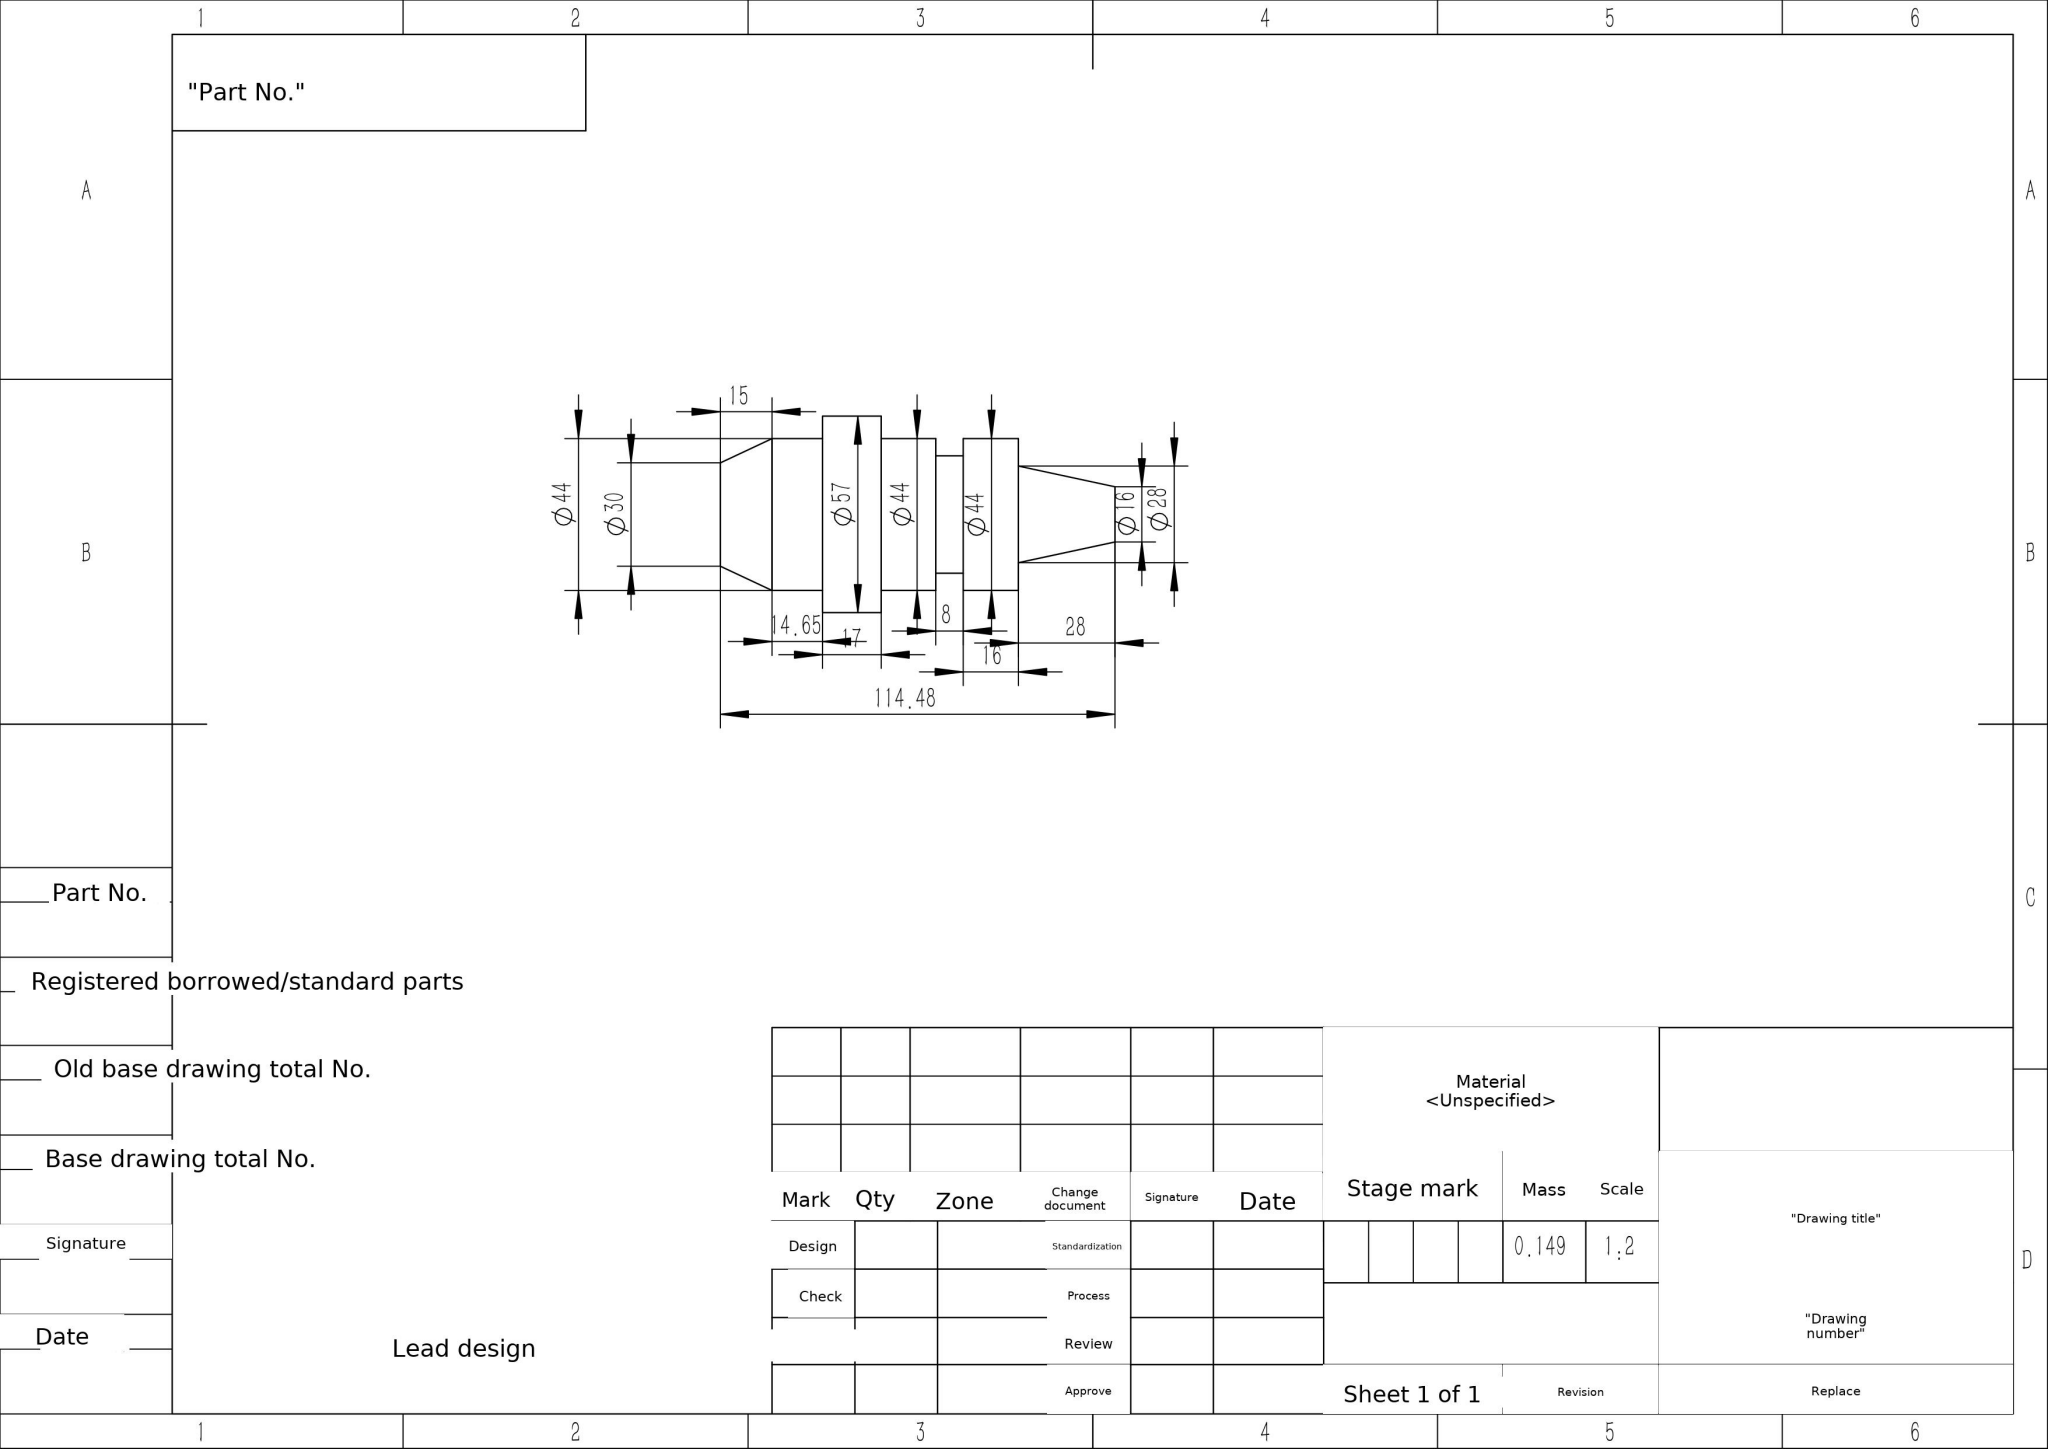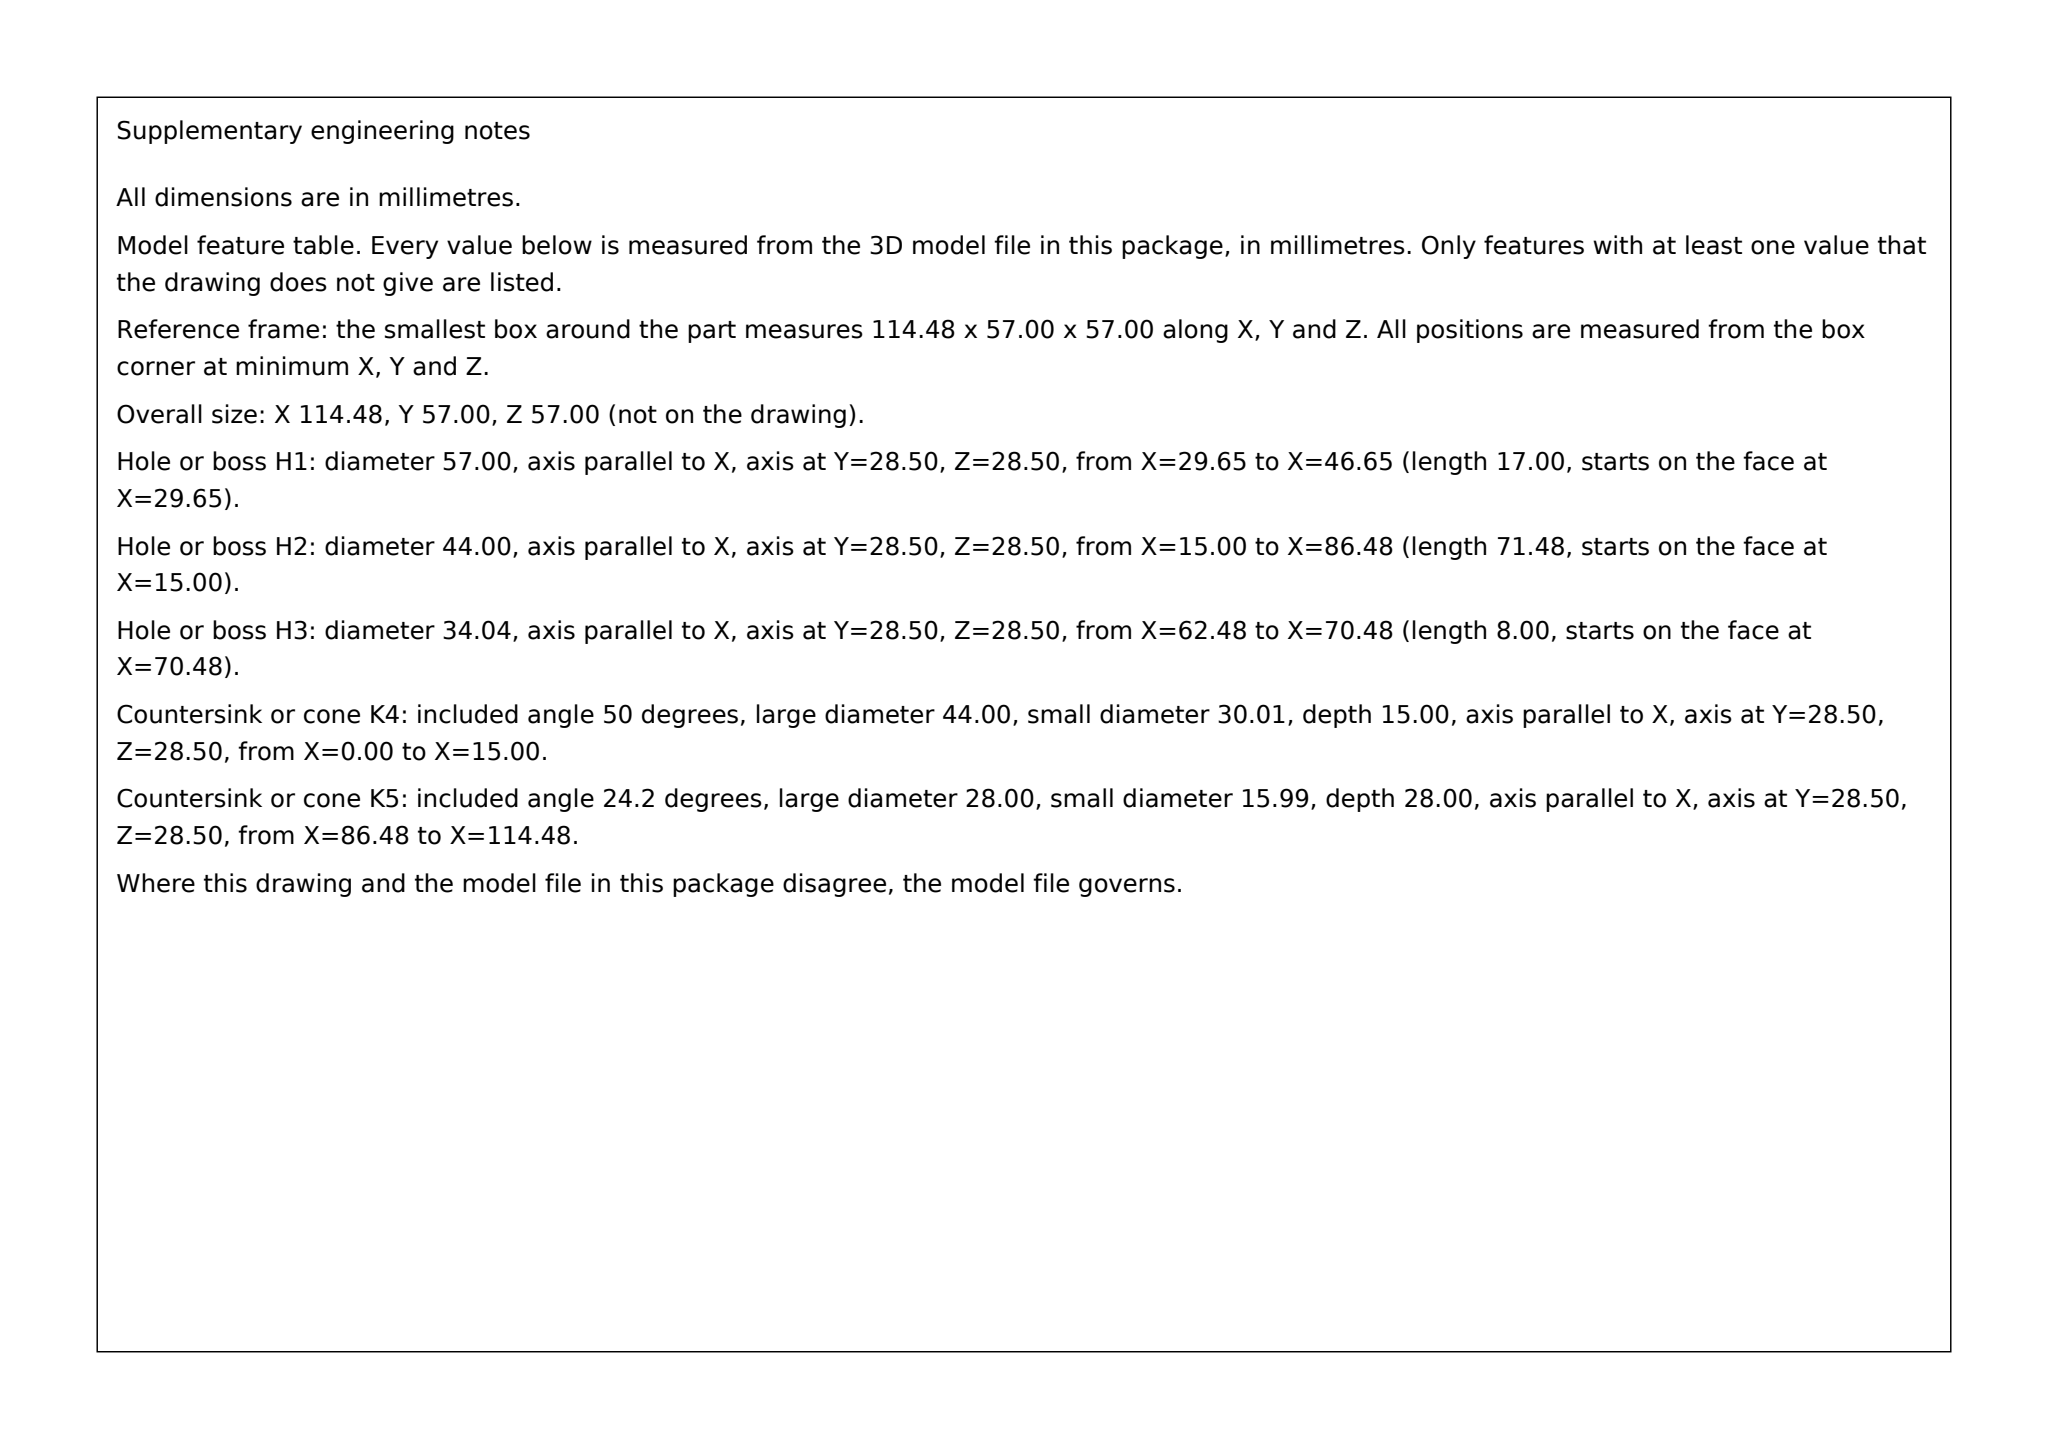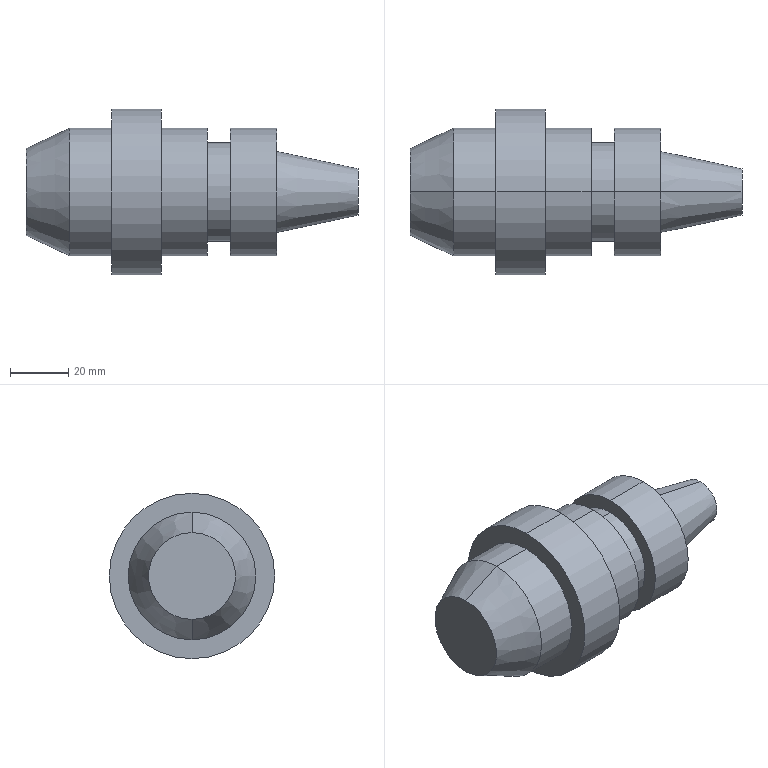Part | SolidWorks | mm | material <Unspecified> | 1 solid | 21 faces | box 114.48 x 57 x 57 mm | volume 148560 mm3 | cylinder 10 | plane 7 | cone 4 | commonest cylinder face diameters 44 x6 34.036 x2 57 x2
build123d program:
from build123d import *


with BuildPart() as part:
    # Sketch1 → Revolve1 (revolve)
    with BuildSketch(Plane.XY, mode=Mode.PRIVATE) as revolve1_sk:
        Polygon((0, 0), (0, 15), (15, 22), (29.653, 22), (29.653, 28.5), (46.653, 28.5), (46.653, 22), (62.479, 22), (62.479, 17.018), (70.479, 17.018), (70.479, 22), (86.479, 22), (86.479, 14), (114.479, 8), (114.479, 0), align=None)
    revolve(revolve1_sk.sketch.rotate(Axis((114.479, 0, 0), (-1, 0, 0)), 90), axis=Axis((114.479, 0, 0), (-1, 0, 0)))


solid = part.part
STEP:
#1=CARTESIAN_POINT('',(114.479,0.,-8.));
#2=VERTEX_POINT('',#1);
#3=CARTESIAN_POINT('',(114.479,0.,8.));
#4=VERTEX_POINT('',#3);
#5=CARTESIAN_POINT('',(114.479,0.,0.));
#6=DIRECTION('',(1.,0.,0.));
#7=DIRECTION('',(0.,0.,-1.));
#8=AXIS2_PLACEMENT_3D('',#5,#6,#7);
#9=CIRCLE('',#8,8.);
#10=EDGE_CURVE('',#2,#4,#9,.T.);
#11=ORIENTED_EDGE('',*,*,#10,.F.);
#12=CARTESIAN_POINT('',(86.479,0.,-14.));
#13=VERTEX_POINT('',#12);
#14=CARTESIAN_POINT('',(114.479,0.,-8.));
#15=DIRECTION('',(-0.9778,0.,-0.2095));
#16=VECTOR('',#15,1000.);
#17=LINE('',#14,#16);
#18=EDGE_CURVE('',#2,#13,#17,.T.);
#19=ORIENTED_EDGE('',*,*,#18,.T.);
#20=CARTESIAN_POINT('',(86.479,0.,14.));
#21=VERTEX_POINT('',#20);
#22=CARTESIAN_POINT('',(86.479,0.,0.));
#23=DIRECTION('',(1.,0.,0.));
#24=DIRECTION('',(0.,0.,-1.));
#25=AXIS2_PLACEMENT_3D('',#22,#23,#24);
#26=CIRCLE('',#25,14.);
#27=EDGE_CURVE('',#13,#21,#26,.T.);
#28=ORIENTED_EDGE('',*,*,#27,.T.);
#29=CARTESIAN_POINT('',(114.479,0.,8.));
#30=DIRECTION('',(-0.9778,0.,0.2095));
#31=VECTOR('',#30,1000.);
#32=LINE('',#29,#31);
#33=EDGE_CURVE('',#4,#21,#32,.T.);
#34=ORIENTED_EDGE('',*,*,#33,.F.);
#35=EDGE_LOOP('',(#11,#19,#28,#34));
#36=FACE_OUTER_BOUND('',#35,.T.);
#37=CARTESIAN_POINT('',(114.479,0.,0.));
#38=DIRECTION('',(-1.,0.,0.));
#39=DIRECTION('',(0.,0.,1.));
#40=AXIS2_PLACEMENT_3D('',#37,#38,#39);
#41=CONICAL_SURFACE('',#40,8.,0.2111);
#42=ADVANCED_FACE('',(#36),#41,.T.);
#43=CARTESIAN_POINT('',(70.479,0.,-22.));
#44=VERTEX_POINT('',#43);
#45=CARTESIAN_POINT('',(70.479,0.,22.));
#46=VERTEX_POINT('',#45);
#47=CARTESIAN_POINT('',(70.479,0.,0.));
#48=DIRECTION('',(1.,0.,0.));
#49=DIRECTION('',(0.,0.,-1.));
#50=AXIS2_PLACEMENT_3D('',#47,#48,#49);
#51=CIRCLE('',#50,22.);
#52=EDGE_CURVE('',#44,#46,#51,.T.);
#53=ORIENTED_EDGE('',*,*,#52,.T.);
#54=CARTESIAN_POINT('',(86.479,0.,22.));
#55=VERTEX_POINT('',#54);
#56=CARTESIAN_POINT('',(114.479,0.,22.));
#57=DIRECTION('',(1.,0.,0.));
#58=VECTOR('',#57,1000.);
#59=LINE('',#56,#58);
#60=EDGE_CURVE('',#46,#55,#59,.T.);
#61=ORIENTED_EDGE('',*,*,#60,.T.);
#62=CARTESIAN_POINT('',(86.479,0.,-22.));
#63=VERTEX_POINT('',#62);
#64=CARTESIAN_POINT('',(86.479,0.,0.));
#65=DIRECTION('',(1.,0.,0.));
#66=DIRECTION('',(0.,0.,-1.));
#67=AXIS2_PLACEMENT_3D('',#64,#65,#66);
#68=CIRCLE('',#67,22.);
#69=EDGE_CURVE('',#63,#55,#68,.T.);
#70=ORIENTED_EDGE('',*,*,#69,.F.);
#71=CARTESIAN_POINT('',(114.479,0.,-22.));
#72=DIRECTION('',(1.,0.,0.));
#73=VECTOR('',#72,1000.);
#74=LINE('',#71,#73);
#75=EDGE_CURVE('',#44,#63,#74,.T.);
#76=ORIENTED_EDGE('',*,*,#75,.F.);
#77=EDGE_LOOP('',(#53,#61,#70,#76));
#78=FACE_OUTER_BOUND('',#77,.T.);
#79=CARTESIAN_POINT('',(114.479,0.,0.));
#80=DIRECTION('',(1.,0.,0.));
#81=DIRECTION('',(0.,0.,-1.));
#82=AXIS2_PLACEMENT_3D('',#79,#80,#81);
#83=CYLINDRICAL_SURFACE('',#82,22.);
#84=ADVANCED_FACE('',(#78),#83,.T.);
#85=CARTESIAN_POINT('',(62.479,0.,-17.018));
#86=VERTEX_POINT('',#85);
#87=CARTESIAN_POINT('',(62.479,0.,17.018));
#88=VERTEX_POINT('',#87);
#89=CARTESIAN_POINT('',(62.479,0.,0.));
#90=DIRECTION('',(1.,0.,0.));
#91=DIRECTION('',(0.,0.,-1.));
#92=AXIS2_PLACEMENT_3D('',#89,#90,#91);
#93=CIRCLE('',#92,17.018);
#94=EDGE_CURVE('',#86,#88,#93,.T.);
#95=ORIENTED_EDGE('',*,*,#94,.T.);
#96=CARTESIAN_POINT('',(70.479,0.,17.018));
#97=VERTEX_POINT('',#96);
#98=CARTESIAN_POINT('',(114.479,0.,17.018));
#99=DIRECTION('',(1.,0.,0.));
#100=VECTOR('',#99,1000.);
#101=LINE('',#98,#100);
#102=EDGE_CURVE('',#88,#97,#101,.T.);
#103=ORIENTED_EDGE('',*,*,#102,.T.);
#104=CARTESIAN_POINT('',(70.479,0.,-17.018));
#105=VERTEX_POINT('',#104);
#106=CARTESIAN_POINT('',(70.479,0.,0.));
#107=DIRECTION('',(1.,0.,0.));
#108=DIRECTION('',(0.,0.,-1.));
#109=AXIS2_PLACEMENT_3D('',#106,#107,#108);
#110=CIRCLE('',#109,17.018);
#111=EDGE_CURVE('',#105,#97,#110,.T.);
#112=ORIENTED_EDGE('',*,*,#111,.F.);
#113=CARTESIAN_POINT('',(114.479,0.,-17.018));
#114=DIRECTION('',(1.,0.,0.));
#115=VECTOR('',#114,1000.);
#116=LINE('',#113,#115);
#117=EDGE_CURVE('',#86,#105,#116,.T.);
#118=ORIENTED_EDGE('',*,*,#117,.F.);
#119=EDGE_LOOP('',(#95,#103,#112,#118));
#120=FACE_OUTER_BOUND('',#119,.T.);
#121=CARTESIAN_POINT('',(114.479,0.,0.));
#122=DIRECTION('',(1.,0.,0.));
#123=DIRECTION('',(0.,0.,-1.));
#124=AXIS2_PLACEMENT_3D('',#121,#122,#123);
#125=CYLINDRICAL_SURFACE('',#124,17.018);
#126=ADVANCED_FACE('',(#120),#125,.T.);
#127=CARTESIAN_POINT('',(46.653,0.,-22.));
#128=VERTEX_POINT('',#127);
#129=CARTESIAN_POINT('',(46.653,0.,22.));
#130=VERTEX_POINT('',#129);
#131=CARTESIAN_POINT('',(46.653,0.,0.));
#132=DIRECTION('',(1.,0.,0.));
#133=DIRECTION('',(0.,0.,-1.));
#134=AXIS2_PLACEMENT_3D('',#131,#132,#133);
#135=CIRCLE('',#134,22.);
#136=EDGE_CURVE('',#128,#130,#135,.T.);
#137=ORIENTED_EDGE('',*,*,#136,.T.);
#138=CARTESIAN_POINT('',(62.479,0.,22.));
#139=VERTEX_POINT('',#138);
#140=CARTESIAN_POINT('',(114.479,0.,22.));
#141=DIRECTION('',(1.,0.,0.));
#142=VECTOR('',#141,1000.);
#143=LINE('',#140,#142);
#144=EDGE_CURVE('',#130,#139,#143,.T.);
#145=ORIENTED_EDGE('',*,*,#144,.T.);
#146=CARTESIAN_POINT('',(62.479,0.,-22.));
#147=VERTEX_POINT('',#146);
#148=CARTESIAN_POINT('',(62.479,0.,0.));
#149=DIRECTION('',(1.,0.,0.));
#150=DIRECTION('',(0.,0.,-1.));
#151=AXIS2_PLACEMENT_3D('',#148,#149,#150);
#152=CIRCLE('',#151,22.);
#153=EDGE_CURVE('',#147,#139,#152,.T.);
#154=ORIENTED_EDGE('',*,*,#153,.F.);
#155=CARTESIAN_POINT('',(114.479,0.,-22.));
#156=DIRECTION('',(1.,0.,0.));
#157=VECTOR('',#156,1000.);
#158=LINE('',#155,#157);
#159=EDGE_CURVE('',#128,#147,#158,.T.);
#160=ORIENTED_EDGE('',*,*,#159,.F.);
#161=EDGE_LOOP('',(#137,#145,#154,#160));
#162=FACE_OUTER_BOUND('',#161,.T.);
#163=CARTESIAN_POINT('',(114.479,0.,0.));
#164=DIRECTION('',(1.,0.,0.));
#165=DIRECTION('',(0.,0.,-1.));
#166=AXIS2_PLACEMENT_3D('',#163,#164,#165);
#167=CYLINDRICAL_SURFACE('',#166,22.);
#168=ADVANCED_FACE('',(#162),#167,.T.);
#169=CARTESIAN_POINT('',(29.653,0.,-28.5));
#170=VERTEX_POINT('',#169);
#171=CARTESIAN_POINT('',(29.653,0.,28.5));
#172=VERTEX_POINT('',#171);
#173=CARTESIAN_POINT('',(29.653,0.,0.));
#174=DIRECTION('',(1.,0.,0.));
#175=DIRECTION('',(0.,0.,-1.));
#176=AXIS2_PLACEMENT_3D('',#173,#174,#175);
#177=CIRCLE('',#176,28.5);
#178=EDGE_CURVE('',#170,#172,#177,.T.);
#179=ORIENTED_EDGE('',*,*,#178,.T.);
#180=CARTESIAN_POINT('',(46.653,0.,28.5));
#181=VERTEX_POINT('',#180);
#182=CARTESIAN_POINT('',(114.479,0.,28.5));
#183=DIRECTION('',(1.,0.,0.));
#184=VECTOR('',#183,1000.);
#185=LINE('',#182,#184);
#186=EDGE_CURVE('',#172,#181,#185,.T.);
#187=ORIENTED_EDGE('',*,*,#186,.T.);
#188=CARTESIAN_POINT('',(46.653,0.,-28.5));
#189=VERTEX_POINT('',#188);
#190=CARTESIAN_POINT('',(46.653,0.,0.));
#191=DIRECTION('',(1.,0.,0.));
#192=DIRECTION('',(0.,0.,-1.));
#193=AXIS2_PLACEMENT_3D('',#190,#191,#192);
#194=CIRCLE('',#193,28.5);
#195=EDGE_CURVE('',#189,#181,#194,.T.);
#196=ORIENTED_EDGE('',*,*,#195,.F.);
#197=CARTESIAN_POINT('',(114.479,0.,-28.5));
#198=DIRECTION('',(1.,0.,0.));
#199=VECTOR('',#198,1000.);
#200=LINE('',#197,#199);
#201=EDGE_CURVE('',#170,#189,#200,.T.);
#202=ORIENTED_EDGE('',*,*,#201,.F.);
#203=EDGE_LOOP('',(#179,#187,#196,#202));
#204=FACE_OUTER_BOUND('',#203,.T.);
#205=CARTESIAN_POINT('',(114.479,0.,0.));
#206=DIRECTION('',(1.,0.,0.));
#207=DIRECTION('',(0.,0.,-1.));
#208=AXIS2_PLACEMENT_3D('',#205,#206,#207);
#209=CYLINDRICAL_SURFACE('',#208,28.5);
#210=ADVANCED_FACE('',(#204),#209,.T.);
#211=CARTESIAN_POINT('',(15.,0.,-22.));
#212=VERTEX_POINT('',#211);
#213=CARTESIAN_POINT('',(15.,0.,22.));
#214=VERTEX_POINT('',#213);
#215=CARTESIAN_POINT('',(15.,0.,0.));
#216=DIRECTION('',(1.,0.,0.));
#217=DIRECTION('',(0.,0.,-1.));
#218=AXIS2_PLACEMENT_3D('',#215,#216,#217);
#219=CIRCLE('',#218,22.);
#220=EDGE_CURVE('',#212,#214,#219,.T.);
#221=ORIENTED_EDGE('',*,*,#220,.T.);
#222=CARTESIAN_POINT('',(29.653,0.,22.));
#223=VERTEX_POINT('',#222);
#224=CARTESIAN_POINT('',(114.479,0.,22.));
#225=DIRECTION('',(1.,0.,0.));
#226=VECTOR('',#225,1000.);
#227=LINE('',#224,#226);
#228=EDGE_CURVE('',#214,#223,#227,.T.);
#229=ORIENTED_EDGE('',*,*,#228,.T.);
#230=CARTESIAN_POINT('',(29.653,0.,-22.));
#231=VERTEX_POINT('',#230);
#232=CARTESIAN_POINT('',(29.653,0.,0.));
#233=DIRECTION('',(1.,0.,0.));
#234=DIRECTION('',(0.,0.,-1.));
#235=AXIS2_PLACEMENT_3D('',#232,#233,#234);
#236=CIRCLE('',#235,22.);
#237=EDGE_CURVE('',#231,#223,#236,.T.);
#238=ORIENTED_EDGE('',*,*,#237,.F.);
#239=CARTESIAN_POINT('',(114.479,0.,-22.));
#240=DIRECTION('',(1.,0.,0.));
#241=VECTOR('',#240,1000.);
#242=LINE('',#239,#241);
#243=EDGE_CURVE('',#212,#231,#242,.T.);
#244=ORIENTED_EDGE('',*,*,#243,.F.);
#245=EDGE_LOOP('',(#221,#229,#238,#244));
#246=FACE_OUTER_BOUND('',#245,.T.);
#247=CARTESIAN_POINT('',(114.479,0.,0.));
#248=DIRECTION('',(1.,0.,0.));
#249=DIRECTION('',(0.,0.,-1.));
#250=AXIS2_PLACEMENT_3D('',#247,#248,#249);
#251=CYLINDRICAL_SURFACE('',#250,22.);
#252=ADVANCED_FACE('',(#246),#251,.T.);
#253=CARTESIAN_POINT('',(0.,0.,-15.));
#254=VERTEX_POINT('',#253);
#255=CARTESIAN_POINT('',(0.,0.,15.));
#256=VERTEX_POINT('',#255);
#257=CARTESIAN_POINT('',(0.,0.,0.));
#258=DIRECTION('',(1.,0.,0.));
#259=DIRECTION('',(0.,0.,-1.));
#260=AXIS2_PLACEMENT_3D('',#257,#258,#259);
#261=CIRCLE('',#260,15.);
#262=EDGE_CURVE('',#254,#256,#261,.T.);
#263=ORIENTED_EDGE('',*,*,#262,.T.);
#264=CARTESIAN_POINT('',(15.,0.,22.));
#265=DIRECTION('',(0.9062,0.,0.4229));
#266=VECTOR('',#265,1000.);
#267=LINE('',#264,#266);
#268=EDGE_CURVE('',#256,#214,#267,.T.);
#269=ORIENTED_EDGE('',*,*,#268,.T.);
#270=ORIENTED_EDGE('',*,*,#220,.F.);
#271=CARTESIAN_POINT('',(15.,0.,-22.));
#272=DIRECTION('',(0.9062,0.,-0.4229));
#273=VECTOR('',#272,1000.);
#274=LINE('',#271,#273);
#275=EDGE_CURVE('',#254,#212,#274,.T.);
#276=ORIENTED_EDGE('',*,*,#275,.F.);
#277=EDGE_LOOP('',(#263,#269,#270,#276));
#278=FACE_OUTER_BOUND('',#277,.T.);
#279=CARTESIAN_POINT('',(15.,0.,0.));
#280=DIRECTION('',(1.,0.,0.));
#281=DIRECTION('',(0.,0.,-1.));
#282=AXIS2_PLACEMENT_3D('',#279,#280,#281);
#283=CONICAL_SURFACE('',#282,22.,0.4366);
#284=ADVANCED_FACE('',(#278),#283,.T.);
#285=ORIENTED_EDGE('',*,*,#262,.F.);
#286=CARTESIAN_POINT('',(0.,0.,0.));
#287=DIRECTION('',(1.,0.,0.));
#288=DIRECTION('',(0.,0.,-1.));
#289=AXIS2_PLACEMENT_3D('',#286,#287,#288);
#290=CIRCLE('',#289,15.);
#291=EDGE_CURVE('',#256,#254,#290,.T.);
#292=ORIENTED_EDGE('',*,*,#291,.F.);
#293=EDGE_LOOP('',(#285,#292));
#294=FACE_OUTER_BOUND('',#293,.T.);
#295=CARTESIAN_POINT('',(0.,0.,0.));
#296=DIRECTION('',(-1.,0.,0.));
#297=DIRECTION('',(0.,0.,1.));
#298=AXIS2_PLACEMENT_3D('',#295,#296,#297);
#299=PLANE('',#298);
#300=ADVANCED_FACE('',(#294),#299,.T.);
#301=ORIENTED_EDGE('',*,*,#268,.F.);
#302=ORIENTED_EDGE('',*,*,#291,.T.);
#303=ORIENTED_EDGE('',*,*,#275,.T.);
#304=CARTESIAN_POINT('',(15.,0.,0.));
#305=DIRECTION('',(1.,0.,0.));
#306=DIRECTION('',(0.,0.,-1.));
#307=AXIS2_PLACEMENT_3D('',#304,#305,#306);
#308=CIRCLE('',#307,22.);
#309=EDGE_CURVE('',#214,#212,#308,.T.);
#310=ORIENTED_EDGE('',*,*,#309,.F.);
#311=EDGE_LOOP('',(#301,#302,#303,#310));
#312=FACE_OUTER_BOUND('',#311,.T.);
#313=CARTESIAN_POINT('',(15.,0.,0.));
#314=DIRECTION('',(1.,0.,0.));
#315=DIRECTION('',(0.,0.,-1.));
#316=AXIS2_PLACEMENT_3D('',#313,#314,#315);
#317=CONICAL_SURFACE('',#316,22.,0.4366);
#318=ADVANCED_FACE('',(#312),#317,.T.);
#319=ORIENTED_EDGE('',*,*,#228,.F.);
#320=ORIENTED_EDGE('',*,*,#309,.T.);
#321=ORIENTED_EDGE('',*,*,#243,.T.);
#322=CARTESIAN_POINT('',(29.653,0.,0.));
#323=DIRECTION('',(1.,0.,0.));
#324=DIRECTION('',(0.,0.,-1.));
#325=AXIS2_PLACEMENT_3D('',#322,#323,#324);
#326=CIRCLE('',#325,22.);
#327=EDGE_CURVE('',#223,#231,#326,.T.);
#328=ORIENTED_EDGE('',*,*,#327,.F.);
#329=EDGE_LOOP('',(#319,#320,#321,#328));
#330=FACE_OUTER_BOUND('',#329,.T.);
#331=CARTESIAN_POINT('',(114.479,0.,0.));
#332=DIRECTION('',(1.,0.,0.));
#333=DIRECTION('',(0.,0.,-1.));
#334=AXIS2_PLACEMENT_3D('',#331,#332,#333);
#335=CYLINDRICAL_SURFACE('',#334,22.);
#336=ADVANCED_FACE('',(#330),#335,.T.);
#337=ORIENTED_EDGE('',*,*,#237,.T.);
#338=ORIENTED_EDGE('',*,*,#327,.T.);
#339=EDGE_LOOP('',(#337,#338));
#340=FACE_BOUND('',#339,.T.);
#341=ORIENTED_EDGE('',*,*,#178,.F.);
#342=CARTESIAN_POINT('',(29.653,0.,0.));
#343=DIRECTION('',(1.,0.,0.));
#344=DIRECTION('',(0.,0.,-1.));
#345=AXIS2_PLACEMENT_3D('',#342,#343,#344);
#346=CIRCLE('',#345,28.5);
#347=EDGE_CURVE('',#172,#170,#346,.T.);
#348=ORIENTED_EDGE('',*,*,#347,.F.);
#349=EDGE_LOOP('',(#341,#348));
#350=FACE_OUTER_BOUND('',#349,.T.);
#351=CARTESIAN_POINT('',(29.653,22.,0.));
#352=DIRECTION('',(-1.,0.,0.));
#353=DIRECTION('',(0.,0.,1.));
#354=AXIS2_PLACEMENT_3D('',#351,#352,#353);
#355=PLANE('',#354);
#356=ADVANCED_FACE('',(#340,#350),#355,.T.);
#357=ORIENTED_EDGE('',*,*,#186,.F.);
#358=ORIENTED_EDGE('',*,*,#347,.T.);
#359=ORIENTED_EDGE('',*,*,#201,.T.);
#360=CARTESIAN_POINT('',(46.653,0.,0.));
#361=DIRECTION('',(1.,0.,0.));
#362=DIRECTION('',(0.,0.,-1.));
#363=AXIS2_PLACEMENT_3D('',#360,#361,#362);
#364=CIRCLE('',#363,28.5);
#365=EDGE_CURVE('',#181,#189,#364,.T.);
#366=ORIENTED_EDGE('',*,*,#365,.F.);
#367=EDGE_LOOP('',(#357,#358,#359,#366));
#368=FACE_OUTER_BOUND('',#367,.T.);
#369=CARTESIAN_POINT('',(114.479,0.,0.));
#370=DIRECTION('',(1.,0.,0.));
#371=DIRECTION('',(0.,0.,-1.));
#372=AXIS2_PLACEMENT_3D('',#369,#370,#371);
#373=CYLINDRICAL_SURFACE('',#372,28.5);
#374=ADVANCED_FACE('',(#368),#373,.T.);
#375=ORIENTED_EDGE('',*,*,#195,.T.);
#376=ORIENTED_EDGE('',*,*,#365,.T.);
#377=EDGE_LOOP('',(#375,#376));
#378=FACE_OUTER_BOUND('',#377,.T.);
#379=ORIENTED_EDGE('',*,*,#136,.F.);
#380=CARTESIAN_POINT('',(46.653,0.,0.));
#381=DIRECTION('',(1.,0.,0.));
#382=DIRECTION('',(0.,0.,-1.));
#383=AXIS2_PLACEMENT_3D('',#380,#381,#382);
#384=CIRCLE('',#383,22.);
#385=EDGE_CURVE('',#130,#128,#384,.T.);
#386=ORIENTED_EDGE('',*,*,#385,.F.);
#387=EDGE_LOOP('',(#379,#386));
#388=FACE_BOUND('',#387,.T.);
#389=CARTESIAN_POINT('',(46.653,28.5,0.));
#390=DIRECTION('',(1.,0.,0.));
#391=DIRECTION('',(0.,0.,-1.));
#392=AXIS2_PLACEMENT_3D('',#389,#390,#391);
#393=PLANE('',#392);
#394=ADVANCED_FACE('',(#378,#388),#393,.T.);
#395=ORIENTED_EDGE('',*,*,#144,.F.);
#396=ORIENTED_EDGE('',*,*,#385,.T.);
#397=ORIENTED_EDGE('',*,*,#159,.T.);
#398=CARTESIAN_POINT('',(62.479,0.,0.));
#399=DIRECTION('',(1.,0.,0.));
#400=DIRECTION('',(0.,0.,-1.));
#401=AXIS2_PLACEMENT_3D('',#398,#399,#400);
#402=CIRCLE('',#401,22.);
#403=EDGE_CURVE('',#139,#147,#402,.T.);
#404=ORIENTED_EDGE('',*,*,#403,.F.);
#405=EDGE_LOOP('',(#395,#396,#397,#404));
#406=FACE_OUTER_BOUND('',#405,.T.);
#407=CARTESIAN_POINT('',(114.479,0.,0.));
#408=DIRECTION('',(1.,0.,0.));
#409=DIRECTION('',(0.,0.,-1.));
#410=AXIS2_PLACEMENT_3D('',#407,#408,#409);
#411=CYLINDRICAL_SURFACE('',#410,22.);
#412=ADVANCED_FACE('',(#406),#411,.T.);
#413=ORIENTED_EDGE('',*,*,#153,.T.);
#414=ORIENTED_EDGE('',*,*,#403,.T.);
#415=EDGE_LOOP('',(#413,#414));
#416=FACE_OUTER_BOUND('',#415,.T.);
#417=ORIENTED_EDGE('',*,*,#94,.F.);
#418=CARTESIAN_POINT('',(62.479,0.,0.));
#419=DIRECTION('',(1.,0.,0.));
#420=DIRECTION('',(0.,0.,-1.));
#421=AXIS2_PLACEMENT_3D('',#418,#419,#420);
#422=CIRCLE('',#421,17.018);
#423=EDGE_CURVE('',#88,#86,#422,.T.);
#424=ORIENTED_EDGE('',*,*,#423,.F.);
#425=EDGE_LOOP('',(#417,#424));
#426=FACE_BOUND('',#425,.T.);
#427=CARTESIAN_POINT('',(62.479,22.,0.));
#428=DIRECTION('',(1.,0.,0.));
#429=DIRECTION('',(0.,0.,-1.));
#430=AXIS2_PLACEMENT_3D('',#427,#428,#429);
#431=PLANE('',#430);
#432=ADVANCED_FACE('',(#416,#426),#431,.T.);
#433=ORIENTED_EDGE('',*,*,#102,.F.);
#434=ORIENTED_EDGE('',*,*,#423,.T.);
#435=ORIENTED_EDGE('',*,*,#117,.T.);
#436=CARTESIAN_POINT('',(70.479,0.,0.));
#437=DIRECTION('',(1.,0.,0.));
#438=DIRECTION('',(0.,0.,-1.));
#439=AXIS2_PLACEMENT_3D('',#436,#437,#438);
#440=CIRCLE('',#439,17.018);
#441=EDGE_CURVE('',#97,#105,#440,.T.);
#442=ORIENTED_EDGE('',*,*,#441,.F.);
#443=EDGE_LOOP('',(#433,#434,#435,#442));
#444=FACE_OUTER_BOUND('',#443,.T.);
#445=CARTESIAN_POINT('',(114.479,0.,0.));
#446=DIRECTION('',(1.,0.,0.));
#447=DIRECTION('',(0.,0.,-1.));
#448=AXIS2_PLACEMENT_3D('',#445,#446,#447);
#449=CYLINDRICAL_SURFACE('',#448,17.018);
#450=ADVANCED_FACE('',(#444),#449,.T.);
#451=ORIENTED_EDGE('',*,*,#111,.T.);
#452=ORIENTED_EDGE('',*,*,#441,.T.);
#453=EDGE_LOOP('',(#451,#452));
#454=FACE_BOUND('',#453,.T.);
#455=ORIENTED_EDGE('',*,*,#52,.F.);
#456=CARTESIAN_POINT('',(70.479,0.,0.));
#457=DIRECTION('',(1.,0.,0.));
#458=DIRECTION('',(0.,0.,-1.));
#459=AXIS2_PLACEMENT_3D('',#456,#457,#458);
#460=CIRCLE('',#459,22.);
#461=EDGE_CURVE('',#46,#44,#460,.T.);
#462=ORIENTED_EDGE('',*,*,#461,.F.);
#463=EDGE_LOOP('',(#455,#462));
#464=FACE_OUTER_BOUND('',#463,.T.);
#465=CARTESIAN_POINT('',(70.479,17.018,0.));
#466=DIRECTION('',(-1.,0.,0.));
#467=DIRECTION('',(0.,0.,1.));
#468=AXIS2_PLACEMENT_3D('',#465,#466,#467);
#469=PLANE('',#468);
#470=ADVANCED_FACE('',(#454,#464),#469,.T.);
#471=ORIENTED_EDGE('',*,*,#60,.F.);
#472=ORIENTED_EDGE('',*,*,#461,.T.);
#473=ORIENTED_EDGE('',*,*,#75,.T.);
#474=CARTESIAN_POINT('',(86.479,0.,0.));
#475=DIRECTION('',(1.,0.,0.));
#476=DIRECTION('',(0.,0.,-1.));
#477=AXIS2_PLACEMENT_3D('',#474,#475,#476);
#478=CIRCLE('',#477,22.);
#479=EDGE_CURVE('',#55,#63,#478,.T.);
#480=ORIENTED_EDGE('',*,*,#479,.F.);
#481=EDGE_LOOP('',(#471,#472,#473,#480));
#482=FACE_OUTER_BOUND('',#481,.T.);
#483=CARTESIAN_POINT('',(114.479,0.,0.));
#484=DIRECTION('',(1.,0.,0.));
#485=DIRECTION('',(0.,0.,-1.));
#486=AXIS2_PLACEMENT_3D('',#483,#484,#485);
#487=CYLINDRICAL_SURFACE('',#486,22.);
#488=ADVANCED_FACE('',(#482),#487,.T.);
#489=ORIENTED_EDGE('',*,*,#69,.T.);
#490=ORIENTED_EDGE('',*,*,#479,.T.);
#491=EDGE_LOOP('',(#489,#490));
#492=FACE_OUTER_BOUND('',#491,.T.);
#493=CARTESIAN_POINT('',(86.479,0.,0.));
#494=DIRECTION('',(1.,0.,0.));
#495=DIRECTION('',(0.,0.,-1.));
#496=AXIS2_PLACEMENT_3D('',#493,#494,#495);
#497=CIRCLE('',#496,14.);
#498=EDGE_CURVE('',#21,#13,#497,.T.);
#499=ORIENTED_EDGE('',*,*,#498,.F.);
#500=ORIENTED_EDGE('',*,*,#27,.F.);
#501=EDGE_LOOP('',(#499,#500));
#502=FACE_BOUND('',#501,.T.);
#503=CARTESIAN_POINT('',(86.479,22.,0.));
#504=DIRECTION('',(1.,0.,0.));
#505=DIRECTION('',(0.,0.,-1.));
#506=AXIS2_PLACEMENT_3D('',#503,#504,#505);
#507=PLANE('',#506);
#508=ADVANCED_FACE('',(#492,#502),#507,.T.);
#509=ORIENTED_EDGE('',*,*,#18,.F.);
#510=CARTESIAN_POINT('',(114.479,0.,0.));
#511=DIRECTION('',(1.,0.,0.));
#512=DIRECTION('',(0.,0.,-1.));
#513=AXIS2_PLACEMENT_3D('',#510,#511,#512);
#514=CIRCLE('',#513,8.);
#515=EDGE_CURVE('',#4,#2,#514,.T.);
#516=ORIENTED_EDGE('',*,*,#515,.F.);
#517=ORIENTED_EDGE('',*,*,#33,.T.);
#518=ORIENTED_EDGE('',*,*,#498,.T.);
#519=EDGE_LOOP('',(#509,#516,#517,#518));
#520=FACE_OUTER_BOUND('',#519,.T.);
#521=CARTESIAN_POINT('',(114.479,0.,0.));
#522=DIRECTION('',(-1.,0.,0.));
#523=DIRECTION('',(0.,0.,1.));
#524=AXIS2_PLACEMENT_3D('',#521,#522,#523);
#525=CONICAL_SURFACE('',#524,8.,0.2111);
#526=ADVANCED_FACE('',(#520),#525,.T.);
#527=ORIENTED_EDGE('',*,*,#515,.T.);
#528=ORIENTED_EDGE('',*,*,#10,.T.);
#529=EDGE_LOOP('',(#527,#528));
#530=FACE_OUTER_BOUND('',#529,.T.);
#531=CARTESIAN_POINT('',(114.479,8.,0.));
#532=DIRECTION('',(1.,0.,0.));
#533=DIRECTION('',(0.,0.,-1.));
#534=AXIS2_PLACEMENT_3D('',#531,#532,#533);
#535=PLANE('',#534);
#536=ADVANCED_FACE('',(#530),#535,.T.);
#537=CLOSED_SHELL('',(#42,#84,#126,#168,#210,#252,#284,#300,#318,#336,#356,#374,#394,#412,#432,#450,#470,#488,#508,#526,#536));
#538=MANIFOLD_SOLID_BREP('',#537);
#539=CARTESIAN_POINT('',(0.,0.,0.));
#540=DIRECTION('',(0.,0.,1.));
#541=DIRECTION('',(1.,0.,0.));
#542=AXIS2_PLACEMENT_3D('',#539,#540,#541);
#543=(LENGTH_UNIT()NAMED_UNIT(*)SI_UNIT(.MILLI.,.METRE.));
#544=UNCERTAINTY_MEASURE_WITH_UNIT(LENGTH_MEASURE(0.00001),#543,'','');
#545=(NAMED_UNIT(*)PLANE_ANGLE_UNIT()SI_UNIT($,.RADIAN.));
#546=(NAMED_UNIT(*)SI_UNIT($,.STERADIAN.)SOLID_ANGLE_UNIT());
#547=(GEOMETRIC_REPRESENTATION_CONTEXT(3)GLOBAL_UNCERTAINTY_ASSIGNED_CONTEXT((#544))GLOBAL_UNIT_ASSIGNED_CONTEXT((#543,#545,#546))REPRESENTATION_CONTEXT('',''));
#548=ADVANCED_BREP_SHAPE_REPRESENTATION('',(#538,#542),#547);